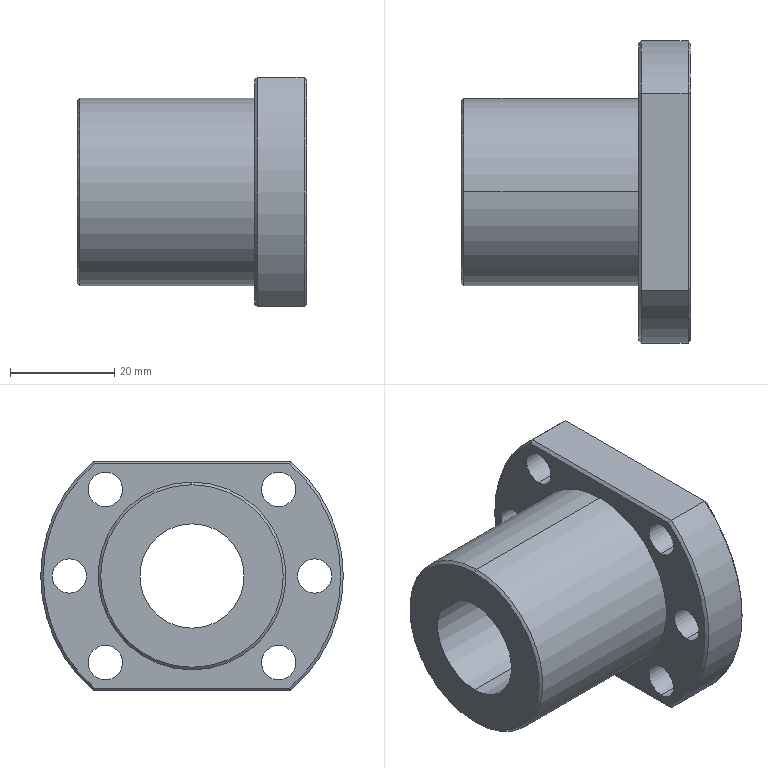Component | SolidWorks | 6G-TL06-Y-AxisMotorAssembly-2_6G-TL06-Y-AxisFlange-1 | 1 solid | 33 faces | box 44 x 58 x 44 mm | volume 41473 mm3 | cylinder 18 | plane 9 | cone 6 | commonest cylinder face diameters 6.6 x12 20 x2 36 x2 58 x2
build123d program:
from build123d import *

# Parameters (mm, degrees)
SKETCH1_R           = 18
BOSS_EXTRUDE1_DEPTH = 34
SKETCH2_R           = 29
BOSS_EXTRUDE2_DEPTH = 10
SKETCH3_R           = 10
CUT_EXTRUDE1_DEPTH  = 61.15
CHAMFER1_SIZE       = 0.5
SKETCH4_R           = 3.3
CUT_EXTRUDE2_DEPTH  = 61.15
SKETCH5_W           = 11.118
SKETCH5_H           = 52.258
SKETCH5_W_2         = 14.394
CUT_EXTRUDE3_DEPTH  = 61.15
CHAMFER2_SIZE       = 0.5


with BuildPart() as part:
    # Sketch1 → Boss-Extrude1 (new body)
    with BuildSketch(Plane.XY):
        Circle(SKETCH1_R)
    extrude(amount=-BOSS_EXTRUDE1_DEPTH)

    # Sketch2 → Boss-Extrude2 (add)
    with BuildSketch(Plane.XY):
        Circle(SKETCH2_R)
    extrude(amount=BOSS_EXTRUDE2_DEPTH)

    # Sketch3 → Cut-Extrude1 (cut, through all)
    with BuildSketch(Plane(origin=(0, 0, -34), x_dir=(-1, 0, 0), z_dir=(0, 0, -1))):
        Circle(SKETCH3_R)
    extrude(amount=-CUT_EXTRUDE1_DEPTH, mode=Mode.SUBTRACT)

    # Chamfer1
    chamfer1_edges = [part.edges().sort_by_distance(p)[0] for p in [
        (-18, 0, -34),
        (-29, 0, 0),
        (-29, 0, 10),
    ]]
    chamfer(chamfer1_edges, length=CHAMFER1_SIZE)

    # Sketch4 → Cut-Extrude2 (cut, through all)
    with BuildSketch(Plane.XY.offset(10)):
        with Locations((-16.617, 16.617)):
            Circle(SKETCH4_R)
        with Locations((0, 23.5)):
            Circle(SKETCH4_R)
        with Locations((16.617, 16.617)):
            Circle(SKETCH4_R)
        with Locations((16.617, -16.617)):
            Circle(SKETCH4_R)
        with Locations((0, -23.5)):
            Circle(SKETCH4_R)
        with Locations((-16.617, -16.617)):
            Circle(SKETCH4_R)
    extrude(amount=-CUT_EXTRUDE2_DEPTH, mode=Mode.SUBTRACT)

    # Sketch5 → Cut-Extrude3 (cut, through all)
    with BuildSketch(Plane.XY.offset(10)):
        with Locations((-27.559, -0.5839)):
            Rectangle(SKETCH5_W, SKETCH5_H)
        with Locations((29.197, -0.5839)):
            Rectangle(SKETCH5_W_2, SKETCH5_H)
    extrude(amount=-CUT_EXTRUDE3_DEPTH, mode=Mode.SUBTRACT)

    # Chamfer2
    chamfer2_edges = [part.edges().sort_by_distance(p)[0] for p in [
        (22, 0, 0),
        (22, 0, 10),
        (-22, 0, 0),
        (-22, 0, 10),
    ]]
    chamfer(chamfer2_edges, length=CHAMFER2_SIZE)


solid = part.part

# Placed as in the assembly
solid = solid.moved(Location((14.036, 0, 20), (0, 90, 0)))
STEP:
#1=CARTESIAN_POINT('',(0.5526,-0.6542,1.572));
#2=VERTEX_POINT('',#1);
#3=CARTESIAN_POINT('',(0.5526,-0.6542,1.312));
#4=VERTEX_POINT('',#3);
#5=CARTESIAN_POINT('',(0.5526,-0.6542,1.442));
#6=DIRECTION('',(1.,0.,-0.));
#7=DIRECTION('',(0.,0.,-1.));
#8=AXIS2_PLACEMENT_3D('',#5,#6,#7);
#9=CIRCLE('',#8,0.1299);
#10=EDGE_CURVE('',#2,#4,#9,.T.);
#11=ORIENTED_EDGE('',*,*,#10,.F.);
#12=CARTESIAN_POINT('',(0.9463,-0.6542,1.572));
#13=VERTEX_POINT('',#12);
#14=CARTESIAN_POINT('',(-0.786,-0.6542,1.572));
#15=DIRECTION('',(1.,0.,-0.));
#16=VECTOR('',#15,39.37);
#17=LINE('',#14,#16);
#18=EDGE_CURVE('',#2,#13,#17,.T.);
#19=ORIENTED_EDGE('',*,*,#18,.T.);
#20=CARTESIAN_POINT('',(0.9463,-0.6542,1.312));
#21=VERTEX_POINT('',#20);
#22=CARTESIAN_POINT('',(0.9463,-0.6542,1.442));
#23=DIRECTION('',(1.,0.,-0.));
#24=DIRECTION('',(0.,0.,-1.));
#25=AXIS2_PLACEMENT_3D('',#22,#23,#24);
#26=CIRCLE('',#25,0.1299);
#27=EDGE_CURVE('',#13,#21,#26,.T.);
#28=ORIENTED_EDGE('',*,*,#27,.T.);
#29=CARTESIAN_POINT('',(-0.786,-0.6542,1.312));
#30=DIRECTION('',(1.,0.,-0.));
#31=VECTOR('',#30,39.37);
#32=LINE('',#29,#31);
#33=EDGE_CURVE('',#4,#21,#32,.T.);
#34=ORIENTED_EDGE('',*,*,#33,.F.);
#35=EDGE_LOOP('',(#11,#19,#28,#34));
#36=FACE_OUTER_BOUND('',#35,.T.);
#37=CARTESIAN_POINT('',(-0.786,-0.6542,1.442));
#38=DIRECTION('',(1.,0.,-0.));
#39=DIRECTION('',(0.,0.,-1.));
#40=AXIS2_PLACEMENT_3D('',#37,#38,#39);
#41=CYLINDRICAL_SURFACE('',#40,0.1299);
#42=ADVANCED_FACE('',(#36),#41,.F.);
#43=CARTESIAN_POINT('',(0.5526,-0.9252,0.9173));
#44=VERTEX_POINT('',#43);
#45=CARTESIAN_POINT('',(0.5526,-0.9252,0.6575));
#46=VERTEX_POINT('',#45);
#47=CARTESIAN_POINT('',(0.5526,-0.9252,0.7874));
#48=DIRECTION('',(1.,0.,-0.));
#49=DIRECTION('',(0.,0.,-1.));
#50=AXIS2_PLACEMENT_3D('',#47,#48,#49);
#51=CIRCLE('',#50,0.1299);
#52=EDGE_CURVE('',#44,#46,#51,.T.);
#53=ORIENTED_EDGE('',*,*,#52,.F.);
#54=CARTESIAN_POINT('',(0.9463,-0.9252,0.9173));
#55=VERTEX_POINT('',#54);
#56=CARTESIAN_POINT('',(-0.786,-0.9252,0.9173));
#57=DIRECTION('',(1.,0.,-0.));
#58=VECTOR('',#57,39.37);
#59=LINE('',#56,#58);
#60=EDGE_CURVE('',#44,#55,#59,.T.);
#61=ORIENTED_EDGE('',*,*,#60,.T.);
#62=CARTESIAN_POINT('',(0.9463,-0.9252,0.6575));
#63=VERTEX_POINT('',#62);
#64=CARTESIAN_POINT('',(0.9463,-0.9252,0.7874));
#65=DIRECTION('',(1.,0.,-0.));
#66=DIRECTION('',(0.,0.,-1.));
#67=AXIS2_PLACEMENT_3D('',#64,#65,#66);
#68=CIRCLE('',#67,0.1299);
#69=EDGE_CURVE('',#55,#63,#68,.T.);
#70=ORIENTED_EDGE('',*,*,#69,.T.);
#71=CARTESIAN_POINT('',(-0.786,-0.9252,0.6575));
#72=DIRECTION('',(1.,0.,-0.));
#73=VECTOR('',#72,39.37);
#74=LINE('',#71,#73);
#75=EDGE_CURVE('',#46,#63,#74,.T.);
#76=ORIENTED_EDGE('',*,*,#75,.F.);
#77=EDGE_LOOP('',(#53,#61,#70,#76));
#78=FACE_OUTER_BOUND('',#77,.T.);
#79=CARTESIAN_POINT('',(-0.786,-0.9252,0.7874));
#80=DIRECTION('',(1.,0.,-0.));
#81=DIRECTION('',(0.,0.,-1.));
#82=AXIS2_PLACEMENT_3D('',#79,#80,#81);
#83=CYLINDRICAL_SURFACE('',#82,0.1299);
#84=ADVANCED_FACE('',(#78),#83,.F.);
#85=CARTESIAN_POINT('',(0.5526,-0.6542,0.2631));
#86=VERTEX_POINT('',#85);
#87=CARTESIAN_POINT('',(0.5526,-0.6542,0.003267));
#88=VERTEX_POINT('',#87);
#89=CARTESIAN_POINT('',(0.5526,-0.6542,0.1332));
#90=DIRECTION('',(1.,0.,-0.));
#91=DIRECTION('',(0.,0.,-1.));
#92=AXIS2_PLACEMENT_3D('',#89,#90,#91);
#93=CIRCLE('',#92,0.1299);
#94=EDGE_CURVE('',#86,#88,#93,.T.);
#95=ORIENTED_EDGE('',*,*,#94,.F.);
#96=CARTESIAN_POINT('',(0.9463,-0.6542,0.2631));
#97=VERTEX_POINT('',#96);
#98=CARTESIAN_POINT('',(-0.786,-0.6542,0.2631));
#99=DIRECTION('',(1.,0.,-0.));
#100=VECTOR('',#99,39.37);
#101=LINE('',#98,#100);
#102=EDGE_CURVE('',#86,#97,#101,.T.);
#103=ORIENTED_EDGE('',*,*,#102,.T.);
#104=CARTESIAN_POINT('',(0.9463,-0.6542,0.003267));
#105=VERTEX_POINT('',#104);
#106=CARTESIAN_POINT('',(0.9463,-0.6542,0.1332));
#107=DIRECTION('',(1.,0.,-0.));
#108=DIRECTION('',(0.,0.,-1.));
#109=AXIS2_PLACEMENT_3D('',#106,#107,#108);
#110=CIRCLE('',#109,0.1299);
#111=EDGE_CURVE('',#97,#105,#110,.T.);
#112=ORIENTED_EDGE('',*,*,#111,.T.);
#113=CARTESIAN_POINT('',(-0.786,-0.6542,0.003267));
#114=DIRECTION('',(1.,0.,-0.));
#115=VECTOR('',#114,39.37);
#116=LINE('',#113,#115);
#117=EDGE_CURVE('',#88,#105,#116,.T.);
#118=ORIENTED_EDGE('',*,*,#117,.F.);
#119=EDGE_LOOP('',(#95,#103,#112,#118));
#120=FACE_OUTER_BOUND('',#119,.T.);
#121=CARTESIAN_POINT('',(-0.786,-0.6542,0.1332));
#122=DIRECTION('',(1.,0.,-0.));
#123=DIRECTION('',(0.,0.,-1.));
#124=AXIS2_PLACEMENT_3D('',#121,#122,#123);
#125=CYLINDRICAL_SURFACE('',#124,0.1299);
#126=ADVANCED_FACE('',(#120),#125,.F.);
#127=CARTESIAN_POINT('',(0.5526,0.6542,0.2631));
#128=VERTEX_POINT('',#127);
#129=CARTESIAN_POINT('',(0.5526,0.6542,0.003267));
#130=VERTEX_POINT('',#129);
#131=CARTESIAN_POINT('',(0.5526,0.6542,0.1332));
#132=DIRECTION('',(1.,0.,-0.));
#133=DIRECTION('',(0.,0.,-1.));
#134=AXIS2_PLACEMENT_3D('',#131,#132,#133);
#135=CIRCLE('',#134,0.1299);
#136=EDGE_CURVE('',#128,#130,#135,.T.);
#137=ORIENTED_EDGE('',*,*,#136,.F.);
#138=CARTESIAN_POINT('',(0.9463,0.6542,0.2631));
#139=VERTEX_POINT('',#138);
#140=CARTESIAN_POINT('',(-0.786,0.6542,0.2631));
#141=DIRECTION('',(1.,0.,-0.));
#142=VECTOR('',#141,39.37);
#143=LINE('',#140,#142);
#144=EDGE_CURVE('',#128,#139,#143,.T.);
#145=ORIENTED_EDGE('',*,*,#144,.T.);
#146=CARTESIAN_POINT('',(0.9463,0.6542,0.003267));
#147=VERTEX_POINT('',#146);
#148=CARTESIAN_POINT('',(0.9463,0.6542,0.1332));
#149=DIRECTION('',(1.,0.,-0.));
#150=DIRECTION('',(0.,0.,-1.));
#151=AXIS2_PLACEMENT_3D('',#148,#149,#150);
#152=CIRCLE('',#151,0.1299);
#153=EDGE_CURVE('',#139,#147,#152,.T.);
#154=ORIENTED_EDGE('',*,*,#153,.T.);
#155=CARTESIAN_POINT('',(-0.786,0.6542,0.003267));
#156=DIRECTION('',(1.,0.,-0.));
#157=VECTOR('',#156,39.37);
#158=LINE('',#155,#157);
#159=EDGE_CURVE('',#130,#147,#158,.T.);
#160=ORIENTED_EDGE('',*,*,#159,.F.);
#161=EDGE_LOOP('',(#137,#145,#154,#160));
#162=FACE_OUTER_BOUND('',#161,.T.);
#163=CARTESIAN_POINT('',(-0.786,0.6542,0.1332));
#164=DIRECTION('',(1.,0.,-0.));
#165=DIRECTION('',(0.,0.,-1.));
#166=AXIS2_PLACEMENT_3D('',#163,#164,#165);
#167=CYLINDRICAL_SURFACE('',#166,0.1299);
#168=ADVANCED_FACE('',(#162),#167,.F.);
#169=CARTESIAN_POINT('',(0.5526,0.9252,0.9173));
#170=VERTEX_POINT('',#169);
#171=CARTESIAN_POINT('',(0.5526,0.9252,0.6575));
#172=VERTEX_POINT('',#171);
#173=CARTESIAN_POINT('',(0.5526,0.9252,0.7874));
#174=DIRECTION('',(1.,0.,-0.));
#175=DIRECTION('',(0.,0.,-1.));
#176=AXIS2_PLACEMENT_3D('',#173,#174,#175);
#177=CIRCLE('',#176,0.1299);
#178=EDGE_CURVE('',#170,#172,#177,.T.);
#179=ORIENTED_EDGE('',*,*,#178,.F.);
#180=CARTESIAN_POINT('',(0.9463,0.9252,0.9173));
#181=VERTEX_POINT('',#180);
#182=CARTESIAN_POINT('',(-0.786,0.9252,0.9173));
#183=DIRECTION('',(1.,0.,-0.));
#184=VECTOR('',#183,39.37);
#185=LINE('',#182,#184);
#186=EDGE_CURVE('',#170,#181,#185,.T.);
#187=ORIENTED_EDGE('',*,*,#186,.T.);
#188=CARTESIAN_POINT('',(0.9463,0.9252,0.6575));
#189=VERTEX_POINT('',#188);
#190=CARTESIAN_POINT('',(0.9463,0.9252,0.7874));
#191=DIRECTION('',(1.,0.,-0.));
#192=DIRECTION('',(0.,0.,-1.));
#193=AXIS2_PLACEMENT_3D('',#190,#191,#192);
#194=CIRCLE('',#193,0.1299);
#195=EDGE_CURVE('',#181,#189,#194,.T.);
#196=ORIENTED_EDGE('',*,*,#195,.T.);
#197=CARTESIAN_POINT('',(-0.786,0.9252,0.6575));
#198=DIRECTION('',(1.,0.,-0.));
#199=VECTOR('',#198,39.37);
#200=LINE('',#197,#199);
#201=EDGE_CURVE('',#172,#189,#200,.T.);
#202=ORIENTED_EDGE('',*,*,#201,.F.);
#203=EDGE_LOOP('',(#179,#187,#196,#202));
#204=FACE_OUTER_BOUND('',#203,.T.);
#205=CARTESIAN_POINT('',(-0.786,0.9252,0.7874));
#206=DIRECTION('',(1.,0.,-0.));
#207=DIRECTION('',(0.,0.,-1.));
#208=AXIS2_PLACEMENT_3D('',#205,#206,#207);
#209=CYLINDRICAL_SURFACE('',#208,0.1299);
#210=ADVANCED_FACE('',(#204),#209,.F.);
#211=CARTESIAN_POINT('',(0.5526,0.6542,1.572));
#212=VERTEX_POINT('',#211);
#213=CARTESIAN_POINT('',(0.5526,0.6542,1.312));
#214=VERTEX_POINT('',#213);
#215=CARTESIAN_POINT('',(0.5526,0.6542,1.442));
#216=DIRECTION('',(1.,0.,-0.));
#217=DIRECTION('',(0.,0.,-1.));
#218=AXIS2_PLACEMENT_3D('',#215,#216,#217);
#219=CIRCLE('',#218,0.1299);
#220=EDGE_CURVE('',#212,#214,#219,.T.);
#221=ORIENTED_EDGE('',*,*,#220,.F.);
#222=CARTESIAN_POINT('',(0.9463,0.6542,1.572));
#223=VERTEX_POINT('',#222);
#224=CARTESIAN_POINT('',(-0.786,0.6542,1.572));
#225=DIRECTION('',(1.,0.,-0.));
#226=VECTOR('',#225,39.37);
#227=LINE('',#224,#226);
#228=EDGE_CURVE('',#212,#223,#227,.T.);
#229=ORIENTED_EDGE('',*,*,#228,.T.);
#230=CARTESIAN_POINT('',(0.9463,0.6542,1.312));
#231=VERTEX_POINT('',#230);
#232=CARTESIAN_POINT('',(0.9463,0.6542,1.442));
#233=DIRECTION('',(1.,0.,-0.));
#234=DIRECTION('',(0.,0.,-1.));
#235=AXIS2_PLACEMENT_3D('',#232,#233,#234);
#236=CIRCLE('',#235,0.1299);
#237=EDGE_CURVE('',#223,#231,#236,.T.);
#238=ORIENTED_EDGE('',*,*,#237,.T.);
#239=CARTESIAN_POINT('',(-0.786,0.6542,1.312));
#240=DIRECTION('',(1.,0.,-0.));
#241=VECTOR('',#240,39.37);
#242=LINE('',#239,#241);
#243=EDGE_CURVE('',#214,#231,#242,.T.);
#244=ORIENTED_EDGE('',*,*,#243,.F.);
#245=EDGE_LOOP('',(#221,#229,#238,#244));
#246=FACE_OUTER_BOUND('',#245,.T.);
#247=CARTESIAN_POINT('',(-0.786,0.6542,1.442));
#248=DIRECTION('',(1.,0.,-0.));
#249=DIRECTION('',(0.,0.,-1.));
#250=AXIS2_PLACEMENT_3D('',#247,#248,#249);
#251=CYLINDRICAL_SURFACE('',#250,0.1299);
#252=ADVANCED_FACE('',(#246),#251,.F.);
#253=CARTESIAN_POINT('',(-0.786,-0.,1.476));
#254=VERTEX_POINT('',#253);
#255=CARTESIAN_POINT('',(-0.786,-0.,0.09843));
#256=VERTEX_POINT('',#255);
#257=CARTESIAN_POINT('',(-0.786,-0.,0.7874));
#258=DIRECTION('',(-1.,-0.,0.));
#259=DIRECTION('',(0.,-0.,-1.));
#260=AXIS2_PLACEMENT_3D('',#257,#258,#259);
#261=CIRCLE('',#260,0.689);
#262=EDGE_CURVE('',#254,#256,#261,.T.);
#263=ORIENTED_EDGE('',*,*,#262,.F.);
#264=CARTESIAN_POINT('',(-0.7663,-0.,1.496));
#265=VERTEX_POINT('',#264);
#266=CARTESIAN_POINT('',(-0.7663,-0.,1.496));
#267=DIRECTION('',(0.7071,0.,0.7071));
#268=VECTOR('',#267,39.37);
#269=LINE('',#266,#268);
#270=EDGE_CURVE('',#254,#265,#269,.T.);
#271=ORIENTED_EDGE('',*,*,#270,.T.);
#272=CARTESIAN_POINT('',(-0.7663,-0.,0.07874));
#273=VERTEX_POINT('',#272);
#274=CARTESIAN_POINT('',(-0.7663,-0.,0.7874));
#275=DIRECTION('',(1.,0.,-0.));
#276=DIRECTION('',(0.,-0.,-1.));
#277=AXIS2_PLACEMENT_3D('',#274,#275,#276);
#278=CIRCLE('',#277,0.7087);
#279=EDGE_CURVE('',#273,#265,#278,.T.);
#280=ORIENTED_EDGE('',*,*,#279,.F.);
#281=CARTESIAN_POINT('',(-0.7663,-0.,0.07874));
#282=DIRECTION('',(0.7071,-0.,-0.7071));
#283=VECTOR('',#282,39.37);
#284=LINE('',#281,#283);
#285=EDGE_CURVE('',#256,#273,#284,.T.);
#286=ORIENTED_EDGE('',*,*,#285,.F.);
#287=EDGE_LOOP('',(#263,#271,#280,#286));
#288=FACE_OUTER_BOUND('',#287,.T.);
#289=CARTESIAN_POINT('',(-0.7663,-0.,0.7874));
#290=DIRECTION('',(1.,0.,-0.));
#291=DIRECTION('',(0.,-0.,-1.));
#292=AXIS2_PLACEMENT_3D('',#289,#290,#291);
#293=CONICAL_SURFACE('',#292,0.7087,0.7854);
#294=ADVANCED_FACE('',(#288),#293,.T.);
#295=CARTESIAN_POINT('',(0.9463,-0.,0.3937));
#296=VERTEX_POINT('',#295);
#297=CARTESIAN_POINT('',(0.9463,-0.,1.181));
#298=VERTEX_POINT('',#297);
#299=CARTESIAN_POINT('',(0.9463,-0.,0.7874));
#300=DIRECTION('',(-1.,-0.,0.));
#301=DIRECTION('',(0.,0.,1.));
#302=AXIS2_PLACEMENT_3D('',#299,#300,#301);
#303=CIRCLE('',#302,0.3937);
#304=EDGE_CURVE('',#296,#298,#303,.T.);
#305=ORIENTED_EDGE('',*,*,#304,.F.);
#306=CARTESIAN_POINT('',(-0.786,-0.,0.3937));
#307=VERTEX_POINT('',#306);
#308=CARTESIAN_POINT('',(0.9463,-0.,0.3937));
#309=DIRECTION('',(-1.,-0.,0.));
#310=VECTOR('',#309,39.37);
#311=LINE('',#308,#310);
#312=EDGE_CURVE('',#296,#307,#311,.T.);
#313=ORIENTED_EDGE('',*,*,#312,.T.);
#314=CARTESIAN_POINT('',(-0.786,-0.,1.181));
#315=VERTEX_POINT('',#314);
#316=CARTESIAN_POINT('',(-0.786,-0.,0.7874));
#317=DIRECTION('',(-1.,-0.,0.));
#318=DIRECTION('',(0.,0.,1.));
#319=AXIS2_PLACEMENT_3D('',#316,#317,#318);
#320=CIRCLE('',#319,0.3937);
#321=EDGE_CURVE('',#307,#315,#320,.T.);
#322=ORIENTED_EDGE('',*,*,#321,.T.);
#323=CARTESIAN_POINT('',(0.9463,-0.,1.181));
#324=DIRECTION('',(-1.,-0.,0.));
#325=VECTOR('',#324,39.37);
#326=LINE('',#323,#325);
#327=EDGE_CURVE('',#298,#315,#326,.T.);
#328=ORIENTED_EDGE('',*,*,#327,.F.);
#329=EDGE_LOOP('',(#305,#313,#322,#328));
#330=FACE_OUTER_BOUND('',#329,.T.);
#331=CARTESIAN_POINT('',(0.9463,-0.,0.7874));
#332=DIRECTION('',(-1.,-0.,0.));
#333=DIRECTION('',(0.,0.,1.));
#334=AXIS2_PLACEMENT_3D('',#331,#332,#333);
#335=CYLINDRICAL_SURFACE('',#334,0.3937);
#336=ADVANCED_FACE('',(#330),#335,.F.);
#337=ORIENTED_EDGE('',*,*,#279,.T.);
#338=CARTESIAN_POINT('',(0.5526,-0.,1.496));
#339=VERTEX_POINT('',#338);
#340=CARTESIAN_POINT('',(-0.786,-0.,1.496));
#341=DIRECTION('',(1.,0.,-0.));
#342=VECTOR('',#341,39.37);
#343=LINE('',#340,#342);
#344=EDGE_CURVE('',#265,#339,#343,.T.);
#345=ORIENTED_EDGE('',*,*,#344,.T.);
#346=CARTESIAN_POINT('',(0.5526,-0.,0.07874));
#347=VERTEX_POINT('',#346);
#348=CARTESIAN_POINT('',(0.5526,-0.,0.7874));
#349=DIRECTION('',(1.,0.,-0.));
#350=DIRECTION('',(0.,-0.,-1.));
#351=AXIS2_PLACEMENT_3D('',#348,#349,#350);
#352=CIRCLE('',#351,0.7087);
#353=EDGE_CURVE('',#347,#339,#352,.T.);
#354=ORIENTED_EDGE('',*,*,#353,.F.);
#355=CARTESIAN_POINT('',(-0.786,-0.,0.07874));
#356=DIRECTION('',(1.,0.,-0.));
#357=VECTOR('',#356,39.37);
#358=LINE('',#355,#357);
#359=EDGE_CURVE('',#273,#347,#358,.T.);
#360=ORIENTED_EDGE('',*,*,#359,.F.);
#361=EDGE_LOOP('',(#337,#345,#354,#360));
#362=FACE_OUTER_BOUND('',#361,.T.);
#363=CARTESIAN_POINT('',(-0.786,-0.,0.7874));
#364=DIRECTION('',(1.,0.,-0.));
#365=DIRECTION('',(0.,-0.,-1.));
#366=AXIS2_PLACEMENT_3D('',#363,#364,#365);
#367=CYLINDRICAL_SURFACE('',#366,0.7087);
#368=ADVANCED_FACE('',(#362),#367,.T.);
#369=CARTESIAN_POINT('',(0.9266,0.7439,1.654));
#370=VERTEX_POINT('',#369);
#371=CARTESIAN_POINT('',(0.9266,0.7439,-0.07874));
#372=VERTEX_POINT('',#371);
#373=CARTESIAN_POINT('',(0.9266,-0.,0.7874));
#374=DIRECTION('',(-1.,-0.,0.));
#375=DIRECTION('',(0.,-0.,-1.));
#376=AXIS2_PLACEMENT_3D('',#373,#374,#375);
#377=CIRCLE('',#376,1.142);
#378=EDGE_CURVE('',#370,#372,#377,.T.);
#379=ORIENTED_EDGE('',*,*,#378,.T.);
#380=CARTESIAN_POINT('',(0.5723,0.7439,-0.07874));
#381=VERTEX_POINT('',#380);
#382=CARTESIAN_POINT('',(0.9463,0.7439,-0.07874));
#383=DIRECTION('',(-1.,-0.,0.));
#384=VECTOR('',#383,39.37);
#385=LINE('',#382,#384);
#386=EDGE_CURVE('',#372,#381,#385,.T.);
#387=ORIENTED_EDGE('',*,*,#386,.T.);
#388=CARTESIAN_POINT('',(0.5723,0.7439,1.654));
#389=VERTEX_POINT('',#388);
#390=CARTESIAN_POINT('',(0.5723,-0.,0.7874));
#391=DIRECTION('',(1.,0.,-0.));
#392=DIRECTION('',(0.,-0.,-1.));
#393=AXIS2_PLACEMENT_3D('',#390,#391,#392);
#394=CIRCLE('',#393,1.142);
#395=EDGE_CURVE('',#381,#389,#394,.T.);
#396=ORIENTED_EDGE('',*,*,#395,.T.);
#397=CARTESIAN_POINT('',(0.9463,0.7439,1.654));
#398=DIRECTION('',(1.,0.,-0.));
#399=VECTOR('',#398,39.37);
#400=LINE('',#397,#399);
#401=EDGE_CURVE('',#389,#370,#400,.T.);
#402=ORIENTED_EDGE('',*,*,#401,.T.);
#403=EDGE_LOOP('',(#379,#387,#396,#402));
#404=FACE_OUTER_BOUND('',#403,.T.);
#405=CARTESIAN_POINT('',(0.9463,-0.,0.7874));
#406=DIRECTION('',(-1.,-0.,0.));
#407=DIRECTION('',(0.,0.,1.));
#408=AXIS2_PLACEMENT_3D('',#405,#406,#407);
#409=CYLINDRICAL_SURFACE('',#408,1.142);
#410=ADVANCED_FACE('',(#404),#409,.T.);
#411=CARTESIAN_POINT('',(0.9463,0.7365,-0.05906));
#412=VERTEX_POINT('',#411);
#413=CARTESIAN_POINT('',(0.9463,0.7365,1.634));
#414=VERTEX_POINT('',#413);
#415=CARTESIAN_POINT('',(0.9463,-0.,0.7874));
#416=DIRECTION('',(1.,0.,-0.));
#417=DIRECTION('',(0.,-0.,-1.));
#418=AXIS2_PLACEMENT_3D('',#415,#416,#417);
#419=CIRCLE('',#418,1.122);
#420=EDGE_CURVE('',#412,#414,#419,.T.);
#421=ORIENTED_EDGE('',*,*,#420,.F.);
#422=CARTESIAN_POINT('',(0.9463,0.7365,-0.05906));
#423=CARTESIAN_POINT('',(0.9397,0.739,-0.06561));
#424=CARTESIAN_POINT('',(0.9332,0.7414,-0.07218));
#425=CARTESIAN_POINT('',(0.9266,0.7439,-0.07874));
#426=B_SPLINE_CURVE_WITH_KNOTS('',3,(#422,#423,#424,#425),.UNSPECIFIED.,.F.,.F.,(4,4),(0.,0.0007312),.UNSPECIFIED.);
#427=EDGE_CURVE('',#412,#372,#426,.T.);
#428=ORIENTED_EDGE('',*,*,#427,.T.);
#429=ORIENTED_EDGE('',*,*,#378,.F.);
#430=CARTESIAN_POINT('',(0.9266,0.7439,1.654));
#431=CARTESIAN_POINT('',(0.9332,0.7414,1.647));
#432=CARTESIAN_POINT('',(0.9397,0.739,1.64));
#433=CARTESIAN_POINT('',(0.9463,0.7365,1.634));
#434=B_SPLINE_CURVE_WITH_KNOTS('',3,(#430,#431,#432,#433),.UNSPECIFIED.,.F.,.F.,(4,4),(0.,0.0007312),.UNSPECIFIED.);
#435=EDGE_CURVE('',#370,#414,#434,.T.);
#436=ORIENTED_EDGE('',*,*,#435,.T.);
#437=EDGE_LOOP('',(#421,#428,#429,#436));
#438=FACE_OUTER_BOUND('',#437,.T.);
#439=CARTESIAN_POINT('',(0.9463,-0.,0.7874));
#440=DIRECTION('',(-1.,-0.,0.));
#441=DIRECTION('',(0.,0.,1.));
#442=AXIS2_PLACEMENT_3D('',#439,#440,#441);
#443=CONICAL_SURFACE('',#442,1.122,0.7854);
#444=ADVANCED_FACE('',(#438),#443,.T.);
#445=CARTESIAN_POINT('',(0.5526,-0.7365,-0.05906));
#446=VERTEX_POINT('',#445);
#447=CARTESIAN_POINT('',(0.5526,-0.7365,1.634));
#448=VERTEX_POINT('',#447);
#449=CARTESIAN_POINT('',(0.5526,-0.,0.7874));
#450=DIRECTION('',(-1.,-0.,0.));
#451=DIRECTION('',(0.,-0.,-1.));
#452=AXIS2_PLACEMENT_3D('',#449,#450,#451);
#453=CIRCLE('',#452,1.122);
#454=EDGE_CURVE('',#446,#448,#453,.T.);
#455=ORIENTED_EDGE('',*,*,#454,.F.);
#456=CARTESIAN_POINT('',(0.5723,-0.7439,-0.07874));
#457=VERTEX_POINT('',#456);
#458=CARTESIAN_POINT('',(0.5526,-0.7365,-0.05906));
#459=CARTESIAN_POINT('',(0.5592,-0.739,-0.06561));
#460=CARTESIAN_POINT('',(0.5657,-0.7414,-0.07218));
#461=CARTESIAN_POINT('',(0.5723,-0.7439,-0.07874));
#462=B_SPLINE_CURVE_WITH_KNOTS('',3,(#458,#459,#460,#461),.UNSPECIFIED.,.F.,.F.,(4,4),(0.,0.0007312),.UNSPECIFIED.);
#463=EDGE_CURVE('',#446,#457,#462,.T.);
#464=ORIENTED_EDGE('',*,*,#463,.T.);
#465=CARTESIAN_POINT('',(0.5723,-0.7439,1.654));
#466=VERTEX_POINT('',#465);
#467=CARTESIAN_POINT('',(0.5723,-0.,0.7874));
#468=DIRECTION('',(1.,0.,-0.));
#469=DIRECTION('',(0.,-0.,-1.));
#470=AXIS2_PLACEMENT_3D('',#467,#468,#469);
#471=CIRCLE('',#470,1.142);
#472=EDGE_CURVE('',#466,#457,#471,.T.);
#473=ORIENTED_EDGE('',*,*,#472,.F.);
#474=CARTESIAN_POINT('',(0.5723,-0.7439,1.654));
#475=CARTESIAN_POINT('',(0.5657,-0.7414,1.647));
#476=CARTESIAN_POINT('',(0.5592,-0.739,1.64));
#477=CARTESIAN_POINT('',(0.5526,-0.7365,1.634));
#478=B_SPLINE_CURVE_WITH_KNOTS('',3,(#474,#475,#476,#477),.UNSPECIFIED.,.F.,.F.,(4,4),(0.,0.0007312),.UNSPECIFIED.);
#479=EDGE_CURVE('',#466,#448,#478,.T.);
#480=ORIENTED_EDGE('',*,*,#479,.T.);
#481=EDGE_LOOP('',(#455,#464,#473,#480));
#482=FACE_OUTER_BOUND('',#481,.T.);
#483=CARTESIAN_POINT('',(0.5723,-0.,0.7874));
#484=DIRECTION('',(1.,0.,-0.));
#485=DIRECTION('',(0.,-0.,-1.));
#486=AXIS2_PLACEMENT_3D('',#483,#484,#485);
#487=CONICAL_SURFACE('',#486,1.142,0.7854);
#488=ADVANCED_FACE('',(#482),#487,.T.);
#489=ORIENTED_EDGE('',*,*,#344,.F.);
#490=CARTESIAN_POINT('',(-0.7663,-0.,0.7874));
#491=DIRECTION('',(1.,0.,-0.));
#492=DIRECTION('',(0.,-0.,-1.));
#493=AXIS2_PLACEMENT_3D('',#490,#491,#492);
#494=CIRCLE('',#493,0.7087);
#495=EDGE_CURVE('',#265,#273,#494,.T.);
#496=ORIENTED_EDGE('',*,*,#495,.T.);
#497=ORIENTED_EDGE('',*,*,#359,.T.);
#498=CARTESIAN_POINT('',(0.5526,-0.,0.7874));
#499=DIRECTION('',(1.,0.,-0.));
#500=DIRECTION('',(0.,-0.,-1.));
#501=AXIS2_PLACEMENT_3D('',#498,#499,#500);
#502=CIRCLE('',#501,0.7087);
#503=EDGE_CURVE('',#339,#347,#502,.T.);
#504=ORIENTED_EDGE('',*,*,#503,.F.);
#505=EDGE_LOOP('',(#489,#496,#497,#504));
#506=FACE_OUTER_BOUND('',#505,.T.);
#507=CARTESIAN_POINT('',(-0.786,-0.,0.7874));
#508=DIRECTION('',(1.,0.,-0.));
#509=DIRECTION('',(0.,-0.,-1.));
#510=AXIS2_PLACEMENT_3D('',#507,#508,#509);
#511=CYLINDRICAL_SURFACE('',#510,0.7087);
#512=ADVANCED_FACE('',(#506),#511,.T.);
#513=CARTESIAN_POINT('',(-0.786,-0.,0.7874));
#514=DIRECTION('',(-1.,-0.,0.));
#515=DIRECTION('',(0.,-0.,-1.));
#516=AXIS2_PLACEMENT_3D('',#513,#514,#515);
#517=CIRCLE('',#516,0.689);
#518=EDGE_CURVE('',#256,#254,#517,.T.);
#519=ORIENTED_EDGE('',*,*,#518,.T.);
#520=ORIENTED_EDGE('',*,*,#262,.T.);
#521=EDGE_LOOP('',(#519,#520));
#522=FACE_OUTER_BOUND('',#521,.T.);
#523=CARTESIAN_POINT('',(-0.786,-0.,0.7874));
#524=DIRECTION('',(-1.,-0.,0.));
#525=DIRECTION('',(0.,0.,1.));
#526=AXIS2_PLACEMENT_3D('',#523,#524,#525);
#527=CIRCLE('',#526,0.3937);
#528=EDGE_CURVE('',#315,#307,#527,.T.);
#529=ORIENTED_EDGE('',*,*,#528,.F.);
#530=ORIENTED_EDGE('',*,*,#321,.F.);
#531=EDGE_LOOP('',(#529,#530));
#532=FACE_BOUND('',#531,.T.);
#533=CARTESIAN_POINT('',(-0.786,-0.,0.7874));
#534=DIRECTION('',(1.,0.,-0.));
#535=DIRECTION('',(-0.,-0.,-1.));
#536=AXIS2_PLACEMENT_3D('',#533,#534,#535);
#537=PLANE('',#536);
#538=ADVANCED_FACE('',(#522,#532),#537,.F.);
#539=ORIENTED_EDGE('',*,*,#472,.T.);
#540=CARTESIAN_POINT('',(0.9266,-0.7439,-0.07874));
#541=VERTEX_POINT('',#540);
#542=CARTESIAN_POINT('',(0.9463,-0.7439,-0.07874));
#543=DIRECTION('',(1.,0.,-0.));
#544=VECTOR('',#543,39.37);
#545=LINE('',#542,#544);
#546=EDGE_CURVE('',#457,#541,#545,.T.);
#547=ORIENTED_EDGE('',*,*,#546,.T.);
#548=CARTESIAN_POINT('',(0.9266,-0.7439,1.654));
#549=VERTEX_POINT('',#548);
#550=CARTESIAN_POINT('',(0.9266,-0.,0.7874));
#551=DIRECTION('',(-1.,-0.,0.));
#552=DIRECTION('',(0.,-0.,-1.));
#553=AXIS2_PLACEMENT_3D('',#550,#551,#552);
#554=CIRCLE('',#553,1.142);
#555=EDGE_CURVE('',#541,#549,#554,.T.);
#556=ORIENTED_EDGE('',*,*,#555,.T.);
#557=CARTESIAN_POINT('',(0.9463,-0.7439,1.654));
#558=DIRECTION('',(-1.,-0.,0.));
#559=VECTOR('',#558,39.37);
#560=LINE('',#557,#559);
#561=EDGE_CURVE('',#549,#466,#560,.T.);
#562=ORIENTED_EDGE('',*,*,#561,.T.);
#563=EDGE_LOOP('',(#539,#547,#556,#562));
#564=FACE_OUTER_BOUND('',#563,.T.);
#565=CARTESIAN_POINT('',(0.9463,-0.,0.7874));
#566=DIRECTION('',(-1.,-0.,0.));
#567=DIRECTION('',(0.,0.,1.));
#568=AXIS2_PLACEMENT_3D('',#565,#566,#567);
#569=CYLINDRICAL_SURFACE('',#568,1.142);
#570=ADVANCED_FACE('',(#564),#569,.T.);
#571=CARTESIAN_POINT('',(0.9463,-0.7365,1.634));
#572=VERTEX_POINT('',#571);
#573=CARTESIAN_POINT('',(0.9463,-0.7365,-0.05906));
#574=VERTEX_POINT('',#573);
#575=CARTESIAN_POINT('',(0.9463,-0.,0.7874));
#576=DIRECTION('',(1.,0.,-0.));
#577=DIRECTION('',(0.,-0.,-1.));
#578=AXIS2_PLACEMENT_3D('',#575,#576,#577);
#579=CIRCLE('',#578,1.122);
#580=EDGE_CURVE('',#572,#574,#579,.T.);
#581=ORIENTED_EDGE('',*,*,#580,.T.);
#582=CARTESIAN_POINT('',(0.9463,0.7133,-0.05906));
#583=DIRECTION('',(-0.,1.,0.));
#584=VECTOR('',#583,39.37);
#585=LINE('',#582,#584);
#586=EDGE_CURVE('',#574,#412,#585,.T.);
#587=ORIENTED_EDGE('',*,*,#586,.T.);
#588=ORIENTED_EDGE('',*,*,#420,.T.);
#589=CARTESIAN_POINT('',(0.9463,-0.7133,1.634));
#590=DIRECTION('',(0.,-1.,-0.));
#591=VECTOR('',#590,39.37);
#592=LINE('',#589,#591);
#593=EDGE_CURVE('',#414,#572,#592,.T.);
#594=ORIENTED_EDGE('',*,*,#593,.T.);
#595=EDGE_LOOP('',(#581,#587,#588,#594));
#596=FACE_OUTER_BOUND('',#595,.T.);
#597=CARTESIAN_POINT('',(0.9463,-0.6542,1.442));
#598=DIRECTION('',(1.,0.,-0.));
#599=DIRECTION('',(0.,0.,-1.));
#600=AXIS2_PLACEMENT_3D('',#597,#598,#599);
#601=CIRCLE('',#600,0.1299);
#602=EDGE_CURVE('',#21,#13,#601,.T.);
#603=ORIENTED_EDGE('',*,*,#602,.F.);
#604=ORIENTED_EDGE('',*,*,#27,.F.);
#605=EDGE_LOOP('',(#603,#604));
#606=FACE_BOUND('',#605,.T.);
#607=CARTESIAN_POINT('',(0.9463,-0.9252,0.7874));
#608=DIRECTION('',(1.,0.,-0.));
#609=DIRECTION('',(0.,0.,-1.));
#610=AXIS2_PLACEMENT_3D('',#607,#608,#609);
#611=CIRCLE('',#610,0.1299);
#612=EDGE_CURVE('',#63,#55,#611,.T.);
#613=ORIENTED_EDGE('',*,*,#612,.F.);
#614=ORIENTED_EDGE('',*,*,#69,.F.);
#615=EDGE_LOOP('',(#613,#614));
#616=FACE_BOUND('',#615,.T.);
#617=CARTESIAN_POINT('',(0.9463,-0.6542,0.1332));
#618=DIRECTION('',(1.,0.,-0.));
#619=DIRECTION('',(0.,0.,-1.));
#620=AXIS2_PLACEMENT_3D('',#617,#618,#619);
#621=CIRCLE('',#620,0.1299);
#622=EDGE_CURVE('',#105,#97,#621,.T.);
#623=ORIENTED_EDGE('',*,*,#622,.F.);
#624=ORIENTED_EDGE('',*,*,#111,.F.);
#625=EDGE_LOOP('',(#623,#624));
#626=FACE_BOUND('',#625,.T.);
#627=CARTESIAN_POINT('',(0.9463,0.6542,0.1332));
#628=DIRECTION('',(1.,0.,-0.));
#629=DIRECTION('',(0.,0.,-1.));
#630=AXIS2_PLACEMENT_3D('',#627,#628,#629);
#631=CIRCLE('',#630,0.1299);
#632=EDGE_CURVE('',#147,#139,#631,.T.);
#633=ORIENTED_EDGE('',*,*,#632,.F.);
#634=ORIENTED_EDGE('',*,*,#153,.F.);
#635=EDGE_LOOP('',(#633,#634));
#636=FACE_BOUND('',#635,.T.);
#637=CARTESIAN_POINT('',(0.9463,0.9252,0.7874));
#638=DIRECTION('',(1.,0.,-0.));
#639=DIRECTION('',(0.,0.,-1.));
#640=AXIS2_PLACEMENT_3D('',#637,#638,#639);
#641=CIRCLE('',#640,0.1299);
#642=EDGE_CURVE('',#189,#181,#641,.T.);
#643=ORIENTED_EDGE('',*,*,#642,.F.);
#644=ORIENTED_EDGE('',*,*,#195,.F.);
#645=EDGE_LOOP('',(#643,#644));
#646=FACE_BOUND('',#645,.T.);
#647=CARTESIAN_POINT('',(0.9463,0.6542,1.442));
#648=DIRECTION('',(1.,0.,-0.));
#649=DIRECTION('',(0.,0.,-1.));
#650=AXIS2_PLACEMENT_3D('',#647,#648,#649);
#651=CIRCLE('',#650,0.1299);
#652=EDGE_CURVE('',#231,#223,#651,.T.);
#653=ORIENTED_EDGE('',*,*,#652,.F.);
#654=ORIENTED_EDGE('',*,*,#237,.F.);
#655=EDGE_LOOP('',(#653,#654));
#656=FACE_BOUND('',#655,.T.);
#657=CARTESIAN_POINT('',(0.9463,-0.,0.7874));
#658=DIRECTION('',(-1.,-0.,0.));
#659=DIRECTION('',(0.,0.,1.));
#660=AXIS2_PLACEMENT_3D('',#657,#658,#659);
#661=CIRCLE('',#660,0.3937);
#662=EDGE_CURVE('',#298,#296,#661,.T.);
#663=ORIENTED_EDGE('',*,*,#662,.T.);
#664=ORIENTED_EDGE('',*,*,#304,.T.);
#665=EDGE_LOOP('',(#663,#664));
#666=FACE_BOUND('',#665,.T.);
#667=CARTESIAN_POINT('',(0.9463,-0.,0.7874));
#668=DIRECTION('',(1.,0.,-0.));
#669=DIRECTION('',(-0.,-0.,-1.));
#670=AXIS2_PLACEMENT_3D('',#667,#668,#669);
#671=PLANE('',#670);
#672=ADVANCED_FACE('',(#596,#606,#616,#626,#636,#646,#656,#666),#671,.T.);
#673=CARTESIAN_POINT('',(0.5526,-0.6542,1.442));
#674=DIRECTION('',(1.,0.,-0.));
#675=DIRECTION('',(0.,0.,-1.));
#676=AXIS2_PLACEMENT_3D('',#673,#674,#675);
#677=CIRCLE('',#676,0.1299);
#678=EDGE_CURVE('',#4,#2,#677,.T.);
#679=ORIENTED_EDGE('',*,*,#678,.T.);
#680=ORIENTED_EDGE('',*,*,#10,.T.);
#681=EDGE_LOOP('',(#679,#680));
#682=FACE_BOUND('',#681,.T.);
#683=CARTESIAN_POINT('',(0.5526,-0.9252,0.7874));
#684=DIRECTION('',(1.,0.,-0.));
#685=DIRECTION('',(0.,0.,-1.));
#686=AXIS2_PLACEMENT_3D('',#683,#684,#685);
#687=CIRCLE('',#686,0.1299);
#688=EDGE_CURVE('',#46,#44,#687,.T.);
#689=ORIENTED_EDGE('',*,*,#688,.T.);
#690=ORIENTED_EDGE('',*,*,#52,.T.);
#691=EDGE_LOOP('',(#689,#690));
#692=FACE_BOUND('',#691,.T.);
#693=CARTESIAN_POINT('',(0.5526,-0.6542,0.1332));
#694=DIRECTION('',(1.,0.,-0.));
#695=DIRECTION('',(0.,0.,-1.));
#696=AXIS2_PLACEMENT_3D('',#693,#694,#695);
#697=CIRCLE('',#696,0.1299);
#698=EDGE_CURVE('',#88,#86,#697,.T.);
#699=ORIENTED_EDGE('',*,*,#698,.T.);
#700=ORIENTED_EDGE('',*,*,#94,.T.);
#701=EDGE_LOOP('',(#699,#700));
#702=FACE_BOUND('',#701,.T.);
#703=CARTESIAN_POINT('',(0.5526,0.6542,0.1332));
#704=DIRECTION('',(1.,0.,-0.));
#705=DIRECTION('',(0.,0.,-1.));
#706=AXIS2_PLACEMENT_3D('',#703,#704,#705);
#707=CIRCLE('',#706,0.1299);
#708=EDGE_CURVE('',#130,#128,#707,.T.);
#709=ORIENTED_EDGE('',*,*,#708,.T.);
#710=ORIENTED_EDGE('',*,*,#136,.T.);
#711=EDGE_LOOP('',(#709,#710));
#712=FACE_BOUND('',#711,.T.);
#713=CARTESIAN_POINT('',(0.5526,0.9252,0.7874));
#714=DIRECTION('',(1.,0.,-0.));
#715=DIRECTION('',(0.,0.,-1.));
#716=AXIS2_PLACEMENT_3D('',#713,#714,#715);
#717=CIRCLE('',#716,0.1299);
#718=EDGE_CURVE('',#172,#170,#717,.T.);
#719=ORIENTED_EDGE('',*,*,#718,.T.);
#720=ORIENTED_EDGE('',*,*,#178,.T.);
#721=EDGE_LOOP('',(#719,#720));
#722=FACE_BOUND('',#721,.T.);
#723=CARTESIAN_POINT('',(0.5526,0.6542,1.442));
#724=DIRECTION('',(1.,0.,-0.));
#725=DIRECTION('',(0.,0.,-1.));
#726=AXIS2_PLACEMENT_3D('',#723,#724,#725);
#727=CIRCLE('',#726,0.1299);
#728=EDGE_CURVE('',#214,#212,#727,.T.);
#729=ORIENTED_EDGE('',*,*,#728,.T.);
#730=ORIENTED_EDGE('',*,*,#220,.T.);
#731=EDGE_LOOP('',(#729,#730));
#732=FACE_BOUND('',#731,.T.);
#733=CARTESIAN_POINT('',(0.5526,0.7365,1.634));
#734=VERTEX_POINT('',#733);
#735=CARTESIAN_POINT('',(0.5526,0.7365,-0.05906));
#736=VERTEX_POINT('',#735);
#737=CARTESIAN_POINT('',(0.5526,-0.,0.7874));
#738=DIRECTION('',(-1.,-0.,0.));
#739=DIRECTION('',(0.,-0.,-1.));
#740=AXIS2_PLACEMENT_3D('',#737,#738,#739);
#741=CIRCLE('',#740,1.122);
#742=EDGE_CURVE('',#734,#736,#741,.T.);
#743=ORIENTED_EDGE('',*,*,#742,.T.);
#744=CARTESIAN_POINT('',(0.5526,-0.,-0.05906));
#745=DIRECTION('',(0.,-1.,-0.));
#746=VECTOR('',#745,39.37);
#747=LINE('',#744,#746);
#748=EDGE_CURVE('',#736,#446,#747,.T.);
#749=ORIENTED_EDGE('',*,*,#748,.T.);
#750=ORIENTED_EDGE('',*,*,#454,.T.);
#751=CARTESIAN_POINT('',(0.5526,-0.,1.634));
#752=DIRECTION('',(-0.,1.,0.));
#753=VECTOR('',#752,39.37);
#754=LINE('',#751,#753);
#755=EDGE_CURVE('',#448,#734,#754,.T.);
#756=ORIENTED_EDGE('',*,*,#755,.T.);
#757=EDGE_LOOP('',(#743,#749,#750,#756));
#758=FACE_OUTER_BOUND('',#757,.T.);
#759=ORIENTED_EDGE('',*,*,#353,.T.);
#760=ORIENTED_EDGE('',*,*,#503,.T.);
#761=EDGE_LOOP('',(#759,#760));
#762=FACE_BOUND('',#761,.T.);
#763=CARTESIAN_POINT('',(0.5526,-0.,0.7874));
#764=DIRECTION('',(1.,0.,-0.));
#765=DIRECTION('',(-0.,-0.,-1.));
#766=AXIS2_PLACEMENT_3D('',#763,#764,#765);
#767=PLANE('',#766);
#768=ADVANCED_FACE('',(#682,#692,#702,#712,#722,#732,#758,#762),#767,.F.);
#769=ORIENTED_EDGE('',*,*,#312,.F.);
#770=ORIENTED_EDGE('',*,*,#662,.F.);
#771=ORIENTED_EDGE('',*,*,#327,.T.);
#772=ORIENTED_EDGE('',*,*,#528,.T.);
#773=EDGE_LOOP('',(#769,#770,#771,#772));
#774=FACE_OUTER_BOUND('',#773,.T.);
#775=CARTESIAN_POINT('',(0.9463,-0.,0.7874));
#776=DIRECTION('',(-1.,-0.,0.));
#777=DIRECTION('',(0.,0.,1.));
#778=AXIS2_PLACEMENT_3D('',#775,#776,#777);
#779=CYLINDRICAL_SURFACE('',#778,0.3937);
#780=ADVANCED_FACE('',(#774),#779,.F.);
#781=ORIENTED_EDGE('',*,*,#270,.F.);
#782=ORIENTED_EDGE('',*,*,#518,.F.);
#783=ORIENTED_EDGE('',*,*,#285,.T.);
#784=ORIENTED_EDGE('',*,*,#495,.F.);
#785=EDGE_LOOP('',(#781,#782,#783,#784));
#786=FACE_OUTER_BOUND('',#785,.T.);
#787=CARTESIAN_POINT('',(-0.7663,-0.,0.7874));
#788=DIRECTION('',(1.,0.,-0.));
#789=DIRECTION('',(0.,-0.,-1.));
#790=AXIS2_PLACEMENT_3D('',#787,#788,#789);
#791=CONICAL_SURFACE('',#790,0.7087,0.7854);
#792=ADVANCED_FACE('',(#786),#791,.T.);
#793=ORIENTED_EDGE('',*,*,#555,.F.);
#794=CARTESIAN_POINT('',(0.9266,-0.7439,-0.07874));
#795=CARTESIAN_POINT('',(0.9332,-0.7414,-0.07218));
#796=CARTESIAN_POINT('',(0.9397,-0.739,-0.06561));
#797=CARTESIAN_POINT('',(0.9463,-0.7365,-0.05906));
#798=B_SPLINE_CURVE_WITH_KNOTS('',3,(#794,#795,#796,#797),.UNSPECIFIED.,.F.,.F.,(4,4),(0.,0.0007312),.UNSPECIFIED.);
#799=EDGE_CURVE('',#541,#574,#798,.T.);
#800=ORIENTED_EDGE('',*,*,#799,.T.);
#801=ORIENTED_EDGE('',*,*,#580,.F.);
#802=CARTESIAN_POINT('',(0.9463,-0.7365,1.634));
#803=CARTESIAN_POINT('',(0.9397,-0.739,1.64));
#804=CARTESIAN_POINT('',(0.9332,-0.7414,1.647));
#805=CARTESIAN_POINT('',(0.9266,-0.7439,1.654));
#806=B_SPLINE_CURVE_WITH_KNOTS('',3,(#802,#803,#804,#805),.UNSPECIFIED.,.F.,.F.,(4,4),(0.,0.0007312),.UNSPECIFIED.);
#807=EDGE_CURVE('',#572,#549,#806,.T.);
#808=ORIENTED_EDGE('',*,*,#807,.T.);
#809=EDGE_LOOP('',(#793,#800,#801,#808));
#810=FACE_OUTER_BOUND('',#809,.T.);
#811=CARTESIAN_POINT('',(0.9463,-0.,0.7874));
#812=DIRECTION('',(-1.,-0.,0.));
#813=DIRECTION('',(0.,0.,1.));
#814=AXIS2_PLACEMENT_3D('',#811,#812,#813);
#815=CONICAL_SURFACE('',#814,1.122,0.7854);
#816=ADVANCED_FACE('',(#810),#815,.T.);
#817=ORIENTED_EDGE('',*,*,#395,.F.);
#818=CARTESIAN_POINT('',(0.5723,0.7439,-0.07874));
#819=CARTESIAN_POINT('',(0.5657,0.7414,-0.07218));
#820=CARTESIAN_POINT('',(0.5592,0.739,-0.06561));
#821=CARTESIAN_POINT('',(0.5526,0.7365,-0.05906));
#822=B_SPLINE_CURVE_WITH_KNOTS('',3,(#818,#819,#820,#821),.UNSPECIFIED.,.F.,.F.,(4,4),(0.,0.0007312),.UNSPECIFIED.);
#823=EDGE_CURVE('',#381,#736,#822,.T.);
#824=ORIENTED_EDGE('',*,*,#823,.T.);
#825=ORIENTED_EDGE('',*,*,#742,.F.);
#826=CARTESIAN_POINT('',(0.5526,0.7365,1.634));
#827=CARTESIAN_POINT('',(0.5592,0.739,1.64));
#828=CARTESIAN_POINT('',(0.5657,0.7414,1.647));
#829=CARTESIAN_POINT('',(0.5723,0.7439,1.654));
#830=B_SPLINE_CURVE_WITH_KNOTS('',3,(#826,#827,#828,#829),.UNSPECIFIED.,.F.,.F.,(4,4),(0.,0.0007312),.UNSPECIFIED.);
#831=EDGE_CURVE('',#734,#389,#830,.T.);
#832=ORIENTED_EDGE('',*,*,#831,.T.);
#833=EDGE_LOOP('',(#817,#824,#825,#832));
#834=FACE_OUTER_BOUND('',#833,.T.);
#835=CARTESIAN_POINT('',(0.5723,-0.,0.7874));
#836=DIRECTION('',(1.,0.,-0.));
#837=DIRECTION('',(0.,-0.,-1.));
#838=AXIS2_PLACEMENT_3D('',#835,#836,#837);
#839=CONICAL_SURFACE('',#838,1.142,0.7854);
#840=ADVANCED_FACE('',(#834),#839,.T.);
#841=ORIENTED_EDGE('',*,*,#228,.F.);
#842=ORIENTED_EDGE('',*,*,#728,.F.);
#843=ORIENTED_EDGE('',*,*,#243,.T.);
#844=ORIENTED_EDGE('',*,*,#652,.T.);
#845=EDGE_LOOP('',(#841,#842,#843,#844));
#846=FACE_OUTER_BOUND('',#845,.T.);
#847=CARTESIAN_POINT('',(-0.786,0.6542,1.442));
#848=DIRECTION('',(1.,0.,-0.));
#849=DIRECTION('',(0.,0.,-1.));
#850=AXIS2_PLACEMENT_3D('',#847,#848,#849);
#851=CYLINDRICAL_SURFACE('',#850,0.1299);
#852=ADVANCED_FACE('',(#846),#851,.F.);
#853=ORIENTED_EDGE('',*,*,#186,.F.);
#854=ORIENTED_EDGE('',*,*,#718,.F.);
#855=ORIENTED_EDGE('',*,*,#201,.T.);
#856=ORIENTED_EDGE('',*,*,#642,.T.);
#857=EDGE_LOOP('',(#853,#854,#855,#856));
#858=FACE_OUTER_BOUND('',#857,.T.);
#859=CARTESIAN_POINT('',(-0.786,0.9252,0.7874));
#860=DIRECTION('',(1.,0.,-0.));
#861=DIRECTION('',(0.,0.,-1.));
#862=AXIS2_PLACEMENT_3D('',#859,#860,#861);
#863=CYLINDRICAL_SURFACE('',#862,0.1299);
#864=ADVANCED_FACE('',(#858),#863,.F.);
#865=ORIENTED_EDGE('',*,*,#144,.F.);
#866=ORIENTED_EDGE('',*,*,#708,.F.);
#867=ORIENTED_EDGE('',*,*,#159,.T.);
#868=ORIENTED_EDGE('',*,*,#632,.T.);
#869=EDGE_LOOP('',(#865,#866,#867,#868));
#870=FACE_OUTER_BOUND('',#869,.T.);
#871=CARTESIAN_POINT('',(-0.786,0.6542,0.1332));
#872=DIRECTION('',(1.,0.,-0.));
#873=DIRECTION('',(0.,0.,-1.));
#874=AXIS2_PLACEMENT_3D('',#871,#872,#873);
#875=CYLINDRICAL_SURFACE('',#874,0.1299);
#876=ADVANCED_FACE('',(#870),#875,.F.);
#877=ORIENTED_EDGE('',*,*,#102,.F.);
#878=ORIENTED_EDGE('',*,*,#698,.F.);
#879=ORIENTED_EDGE('',*,*,#117,.T.);
#880=ORIENTED_EDGE('',*,*,#622,.T.);
#881=EDGE_LOOP('',(#877,#878,#879,#880));
#882=FACE_OUTER_BOUND('',#881,.T.);
#883=CARTESIAN_POINT('',(-0.786,-0.6542,0.1332));
#884=DIRECTION('',(1.,0.,-0.));
#885=DIRECTION('',(0.,0.,-1.));
#886=AXIS2_PLACEMENT_3D('',#883,#884,#885);
#887=CYLINDRICAL_SURFACE('',#886,0.1299);
#888=ADVANCED_FACE('',(#882),#887,.F.);
#889=ORIENTED_EDGE('',*,*,#60,.F.);
#890=ORIENTED_EDGE('',*,*,#688,.F.);
#891=ORIENTED_EDGE('',*,*,#75,.T.);
#892=ORIENTED_EDGE('',*,*,#612,.T.);
#893=EDGE_LOOP('',(#889,#890,#891,#892));
#894=FACE_OUTER_BOUND('',#893,.T.);
#895=CARTESIAN_POINT('',(-0.786,-0.9252,0.7874));
#896=DIRECTION('',(1.,0.,-0.));
#897=DIRECTION('',(0.,0.,-1.));
#898=AXIS2_PLACEMENT_3D('',#895,#896,#897);
#899=CYLINDRICAL_SURFACE('',#898,0.1299);
#900=ADVANCED_FACE('',(#894),#899,.F.);
#901=ORIENTED_EDGE('',*,*,#18,.F.);
#902=ORIENTED_EDGE('',*,*,#678,.F.);
#903=ORIENTED_EDGE('',*,*,#33,.T.);
#904=ORIENTED_EDGE('',*,*,#602,.T.);
#905=EDGE_LOOP('',(#901,#902,#903,#904));
#906=FACE_OUTER_BOUND('',#905,.T.);
#907=CARTESIAN_POINT('',(-0.786,-0.6542,1.442));
#908=DIRECTION('',(1.,0.,-0.));
#909=DIRECTION('',(0.,0.,-1.));
#910=AXIS2_PLACEMENT_3D('',#907,#908,#909);
#911=CYLINDRICAL_SURFACE('',#910,0.1299);
#912=ADVANCED_FACE('',(#906),#911,.F.);
#913=ORIENTED_EDGE('',*,*,#401,.F.);
#914=CARTESIAN_POINT('',(0.5723,1.006,1.654));
#915=DIRECTION('',(0.,-1.,-0.));
#916=VECTOR('',#915,39.37);
#917=LINE('',#914,#916);
#918=EDGE_CURVE('',#389,#466,#917,.T.);
#919=ORIENTED_EDGE('',*,*,#918,.T.);
#920=ORIENTED_EDGE('',*,*,#561,.F.);
#921=CARTESIAN_POINT('',(0.9266,0.7133,1.654));
#922=DIRECTION('',(-0.,1.,0.));
#923=VECTOR('',#922,39.37);
#924=LINE('',#921,#923);
#925=EDGE_CURVE('',#549,#370,#924,.T.);
#926=ORIENTED_EDGE('',*,*,#925,.T.);
#927=EDGE_LOOP('',(#913,#919,#920,#926));
#928=FACE_OUTER_BOUND('',#927,.T.);
#929=CARTESIAN_POINT('',(-0.786,1.006,1.654));
#930=DIRECTION('',(-0.,0.,-1.));
#931=DIRECTION('',(-0.,1.,0.));
#932=AXIS2_PLACEMENT_3D('',#929,#930,#931);
#933=PLANE('',#932);
#934=ADVANCED_FACE('',(#928),#933,.F.);
#935=ORIENTED_EDGE('',*,*,#546,.F.);
#936=CARTESIAN_POINT('',(0.5723,1.006,-0.07874));
#937=DIRECTION('',(-0.,1.,0.));
#938=VECTOR('',#937,39.37);
#939=LINE('',#936,#938);
#940=EDGE_CURVE('',#457,#381,#939,.T.);
#941=ORIENTED_EDGE('',*,*,#940,.T.);
#942=ORIENTED_EDGE('',*,*,#386,.F.);
#943=CARTESIAN_POINT('',(0.9266,-0.7133,-0.07874));
#944=DIRECTION('',(0.,-1.,-0.));
#945=VECTOR('',#944,39.37);
#946=LINE('',#943,#945);
#947=EDGE_CURVE('',#372,#541,#946,.T.);
#948=ORIENTED_EDGE('',*,*,#947,.T.);
#949=EDGE_LOOP('',(#935,#941,#942,#948));
#950=FACE_OUTER_BOUND('',#949,.T.);
#951=CARTESIAN_POINT('',(-0.786,1.006,-0.07874));
#952=DIRECTION('',(0.,-0.,1.));
#953=DIRECTION('',(0.,-1.,-0.));
#954=AXIS2_PLACEMENT_3D('',#951,#952,#953);
#955=PLANE('',#954);
#956=ADVANCED_FACE('',(#950),#955,.F.);
#957=ORIENTED_EDGE('',*,*,#823,.F.);
#958=ORIENTED_EDGE('',*,*,#940,.F.);
#959=ORIENTED_EDGE('',*,*,#463,.F.);
#960=ORIENTED_EDGE('',*,*,#748,.F.);
#961=EDGE_LOOP('',(#957,#958,#959,#960));
#962=FACE_OUTER_BOUND('',#961,.T.);
#963=CARTESIAN_POINT('',(0.5526,-0.,-0.05906));
#964=DIRECTION('',(0.7071,-0.,0.7071));
#965=DIRECTION('',(0.,-1.,-0.));
#966=AXIS2_PLACEMENT_3D('',#963,#964,#965);
#967=PLANE('',#966);
#968=ADVANCED_FACE('',(#962),#967,.F.);
#969=ORIENTED_EDGE('',*,*,#427,.F.);
#970=ORIENTED_EDGE('',*,*,#586,.F.);
#971=ORIENTED_EDGE('',*,*,#799,.F.);
#972=ORIENTED_EDGE('',*,*,#947,.F.);
#973=EDGE_LOOP('',(#969,#970,#971,#972));
#974=FACE_OUTER_BOUND('',#973,.T.);
#975=CARTESIAN_POINT('',(0.9266,1.006,-0.07874));
#976=DIRECTION('',(0.7071,0.,-0.7071));
#977=DIRECTION('',(-0.,1.,0.));
#978=AXIS2_PLACEMENT_3D('',#975,#976,#977);
#979=PLANE('',#978);
#980=ADVANCED_FACE('',(#974),#979,.T.);
#981=ORIENTED_EDGE('',*,*,#479,.F.);
#982=ORIENTED_EDGE('',*,*,#918,.F.);
#983=ORIENTED_EDGE('',*,*,#831,.F.);
#984=ORIENTED_EDGE('',*,*,#755,.F.);
#985=EDGE_LOOP('',(#981,#982,#983,#984));
#986=FACE_OUTER_BOUND('',#985,.T.);
#987=CARTESIAN_POINT('',(0.5526,-0.,1.634));
#988=DIRECTION('',(0.7071,0.,-0.7071));
#989=DIRECTION('',(-0.,1.,0.));
#990=AXIS2_PLACEMENT_3D('',#987,#988,#989);
#991=PLANE('',#990);
#992=ADVANCED_FACE('',(#986),#991,.F.);
#993=ORIENTED_EDGE('',*,*,#807,.F.);
#994=ORIENTED_EDGE('',*,*,#593,.F.);
#995=ORIENTED_EDGE('',*,*,#435,.F.);
#996=ORIENTED_EDGE('',*,*,#925,.F.);
#997=EDGE_LOOP('',(#993,#994,#995,#996));
#998=FACE_OUTER_BOUND('',#997,.T.);
#999=CARTESIAN_POINT('',(0.9266,1.006,1.654));
#1000=DIRECTION('',(0.7071,-0.,0.7071));
#1001=DIRECTION('',(0.,-1.,-0.));
#1002=AXIS2_PLACEMENT_3D('',#999,#1000,#1001);
#1003=PLANE('',#1002);
#1004=ADVANCED_FACE('',(#998),#1003,.T.);
#1005=CLOSED_SHELL('',(#42,#84,#126,#168,#210,#252,#294,#336,#368,#410,#444,#488,#512,#538,#570,#672,#768,#780,#792,#816,#840,#852,#864,#876,#888,#900,#912,#934,#956,#968,#980,#992,#1004));
#1006=MANIFOLD_SOLID_BREP('',#1005);
#1007=CARTESIAN_POINT('',(0.,0.,0.));
#1008=DIRECTION('',(0.,0.,1.));
#1009=DIRECTION('',(1.,0.,0.));
#1010=AXIS2_PLACEMENT_3D('',#1007,#1008,#1009);
#1011=(LENGTH_UNIT()NAMED_UNIT(*)SI_UNIT($,.METRE.));
#1012=LENGTH_MEASURE_WITH_UNIT(LENGTH_MEASURE(0.0254),#1011);
#1013=DIMENSIONAL_EXPONENTS(1.,0.,0.,0.,0.,0.,0.);
#1014=(CONVERSION_BASED_UNIT('',#1012)LENGTH_UNIT()NAMED_UNIT(#1013));
#1015=UNCERTAINTY_MEASURE_WITH_UNIT(LENGTH_MEASURE(0.00001),#1014,'','');
#1016=(NAMED_UNIT(*)PLANE_ANGLE_UNIT()SI_UNIT($,.RADIAN.));
#1017=(NAMED_UNIT(*)SI_UNIT($,.STERADIAN.)SOLID_ANGLE_UNIT());
#1018=(GEOMETRIC_REPRESENTATION_CONTEXT(3)GLOBAL_UNCERTAINTY_ASSIGNED_CONTEXT((#1015))GLOBAL_UNIT_ASSIGNED_CONTEXT((#1014,#1016,#1017))REPRESENTATION_CONTEXT('',''));
#1019=ADVANCED_BREP_SHAPE_REPRESENTATION('',(#1006,#1010),#1018);
#1020=COLOUR_RGB('',0.7922,0.8196,0.9333);
#1021=FILL_AREA_STYLE_COLOUR('',#1020);
#1022=FILL_AREA_STYLE('',(#1021));
#1023=SURFACE_STYLE_FILL_AREA(#1022);
#1024=SURFACE_SIDE_STYLE('',(#1023));
#1025=SURFACE_STYLE_USAGE(.BOTH.,#1024);
#1026=PRESENTATION_STYLE_ASSIGNMENT((#1025));
#1027=STYLED_ITEM('',(#1026),#1006);
#1028=PRESENTATION_LAYER_ASSIGNMENT('','',(#1027));
#1029=(LENGTH_UNIT()NAMED_UNIT(*)SI_UNIT($,.METRE.));
#1030=LENGTH_MEASURE_WITH_UNIT(LENGTH_MEASURE(0.0254),#1029);
#1031=DIMENSIONAL_EXPONENTS(1.,0.,0.,0.,0.,0.,0.);
#1032=(CONVERSION_BASED_UNIT('',#1030)LENGTH_UNIT()NAMED_UNIT(#1031));
#1033=UNCERTAINTY_MEASURE_WITH_UNIT(LENGTH_MEASURE(0.00001),#1032,'','');
#1034=(NAMED_UNIT(*)PLANE_ANGLE_UNIT()SI_UNIT($,.RADIAN.));
#1035=(NAMED_UNIT(*)SI_UNIT($,.STERADIAN.)SOLID_ANGLE_UNIT());
#1036=(GEOMETRIC_REPRESENTATION_CONTEXT(3)GLOBAL_UNCERTAINTY_ASSIGNED_CONTEXT((#1033))GLOBAL_UNIT_ASSIGNED_CONTEXT((#1032,#1034,#1035))REPRESENTATION_CONTEXT('',''));
#1037=MECHANICAL_DESIGN_GEOMETRIC_PRESENTATION_REPRESENTATION('',(#1027),#1036);